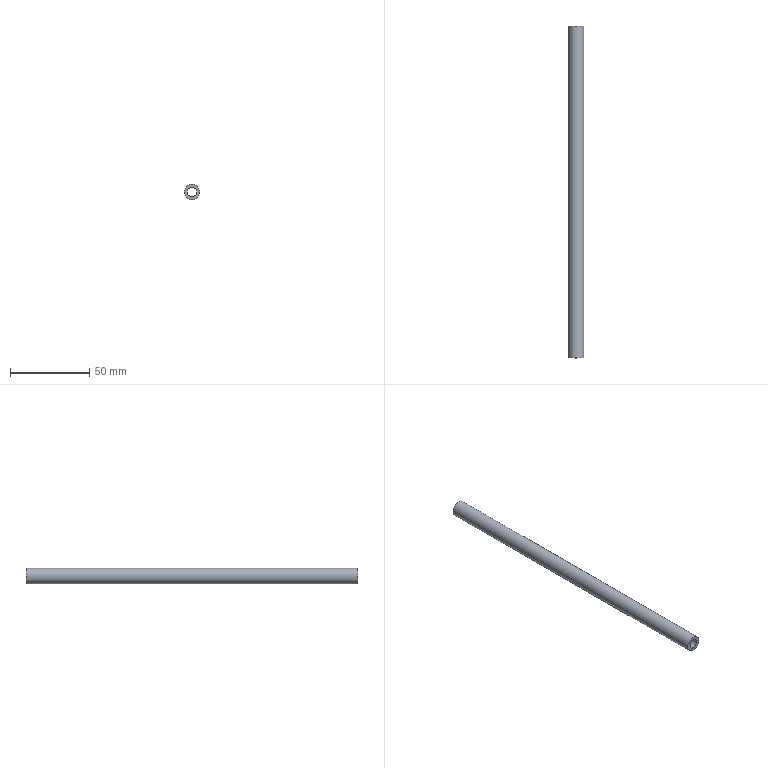Component | NX | CH3404_4-2 | 1 solid | 4 faces | box 10 x 210 x 10 mm | volume 10556 mm3 | cylinder 2 | plane 2 | commonest cylinder face diameters 10 x1 6 x1
STEP:
#1=CARTESIAN_POINT('',(0.,0.,0.));
#2=DIRECTION('',(0.,0.,1.));
#3=DIRECTION('',(1.,0.,0.));
#4=AXIS2_PLACEMENT_3D('',#1,#2,#3);
#5=CARTESIAN_POINT('',(5.,-18.,0.));
#6=VERTEX_POINT('',#5);
#7=CARTESIAN_POINT('',(0.,-18.,0.));
#8=DIRECTION('',(0.,-1.,0.));
#9=DIRECTION('',(1.,0.,0.));
#10=AXIS2_PLACEMENT_3D('',#7,#8,#9);
#11=CIRCLE('',#10,5.);
#12=CARTESIAN_POINT('',(0.,-18.,0.));
#13=DIRECTION('',(0.,1.,0.));
#14=DIRECTION('',(-1.,0.,0.));
#15=AXIS2_PLACEMENT_3D('',#12,#13,#14);
#16=CYLINDRICAL_SURFACE('',#15,5.);
#17=CARTESIAN_POINT('',(9.425,0.));
#18=DIRECTION('',(-1.,0.));
#19=VECTOR('',#18,1.);
#20=LINE('',#17,#19);
#21=(GEOMETRIC_REPRESENTATION_CONTEXT(2)PARAMETRIC_REPRESENTATION_CONTEXT()REPRESENTATION_CONTEXT('',''));
#22=DEFINITIONAL_REPRESENTATION('',(#20),#21);
#23=PCURVE('',#16,#22);
#24=CARTESIAN_POINT('',(0.,-18.,0.));
#25=DIRECTION('',(0.,-1.,0.));
#26=DIRECTION('',(1.,0.,0.));
#27=AXIS2_PLACEMENT_3D('',#24,#25,#26);
#28=PLANE('',#27);
#29=CARTESIAN_POINT('',(0.,0.));
#30=DIRECTION('',(1.,0.));
#31=AXIS2_PLACEMENT_2D('',#29,#30);
#32=CIRCLE('',#31,5.);
#33=(GEOMETRIC_REPRESENTATION_CONTEXT(2)PARAMETRIC_REPRESENTATION_CONTEXT()REPRESENTATION_CONTEXT('',''));
#34=DEFINITIONAL_REPRESENTATION('',(#32),#33);
#35=PCURVE('',#28,#34);
#36=SURFACE_CURVE('',#11,(#23,#35),.PCURVE_S1.);
#37=EDGE_CURVE('',#6,#6,#36,.T.);
#38=ORIENTED_EDGE('',*,*,#37,.F.);
#39=CARTESIAN_POINT('',(5.,192.,0.));
#40=VERTEX_POINT('',#39);
#41=CARTESIAN_POINT('',(5.,-18.,0.));
#42=CARTESIAN_POINT('',(5.,192.,0.));
#43=B_SPLINE_CURVE_WITH_KNOTS('',1,(#41,#42),.UNSPECIFIED.,.F.,.F.,(2,2),(0.,210.),.PIECEWISE_BEZIER_KNOTS.);
#44=CARTESIAN_POINT('',(9.425,0.));
#45=DIRECTION('',(0.,1.));
#46=VECTOR('',#45,1.);
#47=LINE('',#44,#46);
#48=(GEOMETRIC_REPRESENTATION_CONTEXT(2)PARAMETRIC_REPRESENTATION_CONTEXT()REPRESENTATION_CONTEXT('',''));
#49=DEFINITIONAL_REPRESENTATION('',(#47),#48);
#50=PCURVE('',#16,#49);
#51=CARTESIAN_POINT('',(3.142,0.));
#52=DIRECTION('',(0.,1.));
#53=VECTOR('',#52,1.);
#54=LINE('',#51,#53);
#55=(GEOMETRIC_REPRESENTATION_CONTEXT(2)PARAMETRIC_REPRESENTATION_CONTEXT()REPRESENTATION_CONTEXT('',''));
#56=DEFINITIONAL_REPRESENTATION('',(#54),#55);
#57=PCURVE('',#16,#56);
#58=SEAM_CURVE('',#43,(#50,#57),.PCURVE_S1.);
#59=EDGE_CURVE('',#6,#40,#58,.T.);
#60=ORIENTED_EDGE('',*,*,#59,.T.);
#61=CARTESIAN_POINT('',(0.,192.,0.));
#62=DIRECTION('',(0.,-1.,0.));
#63=DIRECTION('',(1.,0.,0.));
#64=AXIS2_PLACEMENT_3D('',#61,#62,#63);
#65=CIRCLE('',#64,5.);
#66=CARTESIAN_POINT('',(9.425,210.));
#67=DIRECTION('',(-1.,0.));
#68=VECTOR('',#67,1.);
#69=LINE('',#66,#68);
#70=(GEOMETRIC_REPRESENTATION_CONTEXT(2)PARAMETRIC_REPRESENTATION_CONTEXT()REPRESENTATION_CONTEXT('',''));
#71=DEFINITIONAL_REPRESENTATION('',(#69),#70);
#72=PCURVE('',#16,#71);
#73=CARTESIAN_POINT('',(0.,192.,0.));
#74=DIRECTION('',(0.,-1.,0.));
#75=DIRECTION('',(1.,0.,0.));
#76=AXIS2_PLACEMENT_3D('',#73,#74,#75);
#77=PLANE('',#76);
#78=CARTESIAN_POINT('',(0.,0.));
#79=DIRECTION('',(1.,0.));
#80=AXIS2_PLACEMENT_2D('',#78,#79);
#81=CIRCLE('',#80,5.);
#82=(GEOMETRIC_REPRESENTATION_CONTEXT(2)PARAMETRIC_REPRESENTATION_CONTEXT()REPRESENTATION_CONTEXT('',''));
#83=DEFINITIONAL_REPRESENTATION('',(#81),#82);
#84=PCURVE('',#77,#83);
#85=SURFACE_CURVE('',#65,(#72,#84),.PCURVE_S1.);
#86=EDGE_CURVE('',#40,#40,#85,.T.);
#87=ORIENTED_EDGE('',*,*,#86,.T.);
#88=ORIENTED_EDGE('',*,*,#59,.F.);
#89=EDGE_LOOP('',(#38,#60,#87,#88));
#90=FACE_BOUND('',#89,.T.);
#91=ADVANCED_FACE('',(#90),#16,.T.);
#92=CARTESIAN_POINT('',(3.,-18.,0.));
#93=VERTEX_POINT('',#92);
#94=CARTESIAN_POINT('',(0.,-18.,0.));
#95=DIRECTION('',(0.,-1.,0.));
#96=DIRECTION('',(1.,0.,0.));
#97=AXIS2_PLACEMENT_3D('',#94,#95,#96);
#98=CIRCLE('',#97,3.);
#99=CARTESIAN_POINT('',(0.,-18.,0.));
#100=DIRECTION('',(0.,1.,0.));
#101=DIRECTION('',(-1.,0.,0.));
#102=AXIS2_PLACEMENT_3D('',#99,#100,#101);
#103=CYLINDRICAL_SURFACE('',#102,3.);
#104=CARTESIAN_POINT('',(9.425,0.));
#105=DIRECTION('',(-1.,0.));
#106=VECTOR('',#105,1.);
#107=LINE('',#104,#106);
#108=(GEOMETRIC_REPRESENTATION_CONTEXT(2)PARAMETRIC_REPRESENTATION_CONTEXT()REPRESENTATION_CONTEXT('',''));
#109=DEFINITIONAL_REPRESENTATION('',(#107),#108);
#110=PCURVE('',#103,#109);
#111=CARTESIAN_POINT('',(0.,0.));
#112=DIRECTION('',(1.,0.));
#113=AXIS2_PLACEMENT_2D('',#111,#112);
#114=CIRCLE('',#113,3.);
#115=(GEOMETRIC_REPRESENTATION_CONTEXT(2)PARAMETRIC_REPRESENTATION_CONTEXT()REPRESENTATION_CONTEXT('',''));
#116=DEFINITIONAL_REPRESENTATION('',(#114),#115);
#117=PCURVE('',#28,#116);
#118=SURFACE_CURVE('',#98,(#110,#117),.PCURVE_S1.);
#119=EDGE_CURVE('',#93,#93,#118,.T.);
#120=ORIENTED_EDGE('',*,*,#119,.F.);
#121=CARTESIAN_POINT('',(3.,192.,0.));
#122=VERTEX_POINT('',#121);
#123=CARTESIAN_POINT('',(3.,-18.,0.));
#124=CARTESIAN_POINT('',(3.,192.,0.));
#125=B_SPLINE_CURVE_WITH_KNOTS('',1,(#123,#124),.UNSPECIFIED.,.F.,.F.,(2,2),(0.,210.),.PIECEWISE_BEZIER_KNOTS.);
#126=CARTESIAN_POINT('',(9.425,0.));
#127=DIRECTION('',(0.,1.));
#128=VECTOR('',#127,1.);
#129=LINE('',#126,#128);
#130=(GEOMETRIC_REPRESENTATION_CONTEXT(2)PARAMETRIC_REPRESENTATION_CONTEXT()REPRESENTATION_CONTEXT('',''));
#131=DEFINITIONAL_REPRESENTATION('',(#129),#130);
#132=PCURVE('',#103,#131);
#133=CARTESIAN_POINT('',(3.142,0.));
#134=DIRECTION('',(0.,1.));
#135=VECTOR('',#134,1.);
#136=LINE('',#133,#135);
#137=(GEOMETRIC_REPRESENTATION_CONTEXT(2)PARAMETRIC_REPRESENTATION_CONTEXT()REPRESENTATION_CONTEXT('',''));
#138=DEFINITIONAL_REPRESENTATION('',(#136),#137);
#139=PCURVE('',#103,#138);
#140=SEAM_CURVE('',#125,(#132,#139),.PCURVE_S1.);
#141=EDGE_CURVE('',#93,#122,#140,.T.);
#142=ORIENTED_EDGE('',*,*,#141,.T.);
#143=CARTESIAN_POINT('',(0.,192.,0.));
#144=DIRECTION('',(0.,-1.,0.));
#145=DIRECTION('',(1.,0.,0.));
#146=AXIS2_PLACEMENT_3D('',#143,#144,#145);
#147=CIRCLE('',#146,3.);
#148=CARTESIAN_POINT('',(9.425,210.));
#149=DIRECTION('',(-1.,0.));
#150=VECTOR('',#149,1.);
#151=LINE('',#148,#150);
#152=(GEOMETRIC_REPRESENTATION_CONTEXT(2)PARAMETRIC_REPRESENTATION_CONTEXT()REPRESENTATION_CONTEXT('',''));
#153=DEFINITIONAL_REPRESENTATION('',(#151),#152);
#154=PCURVE('',#103,#153);
#155=CARTESIAN_POINT('',(0.,0.));
#156=DIRECTION('',(1.,0.));
#157=AXIS2_PLACEMENT_2D('',#155,#156);
#158=CIRCLE('',#157,3.);
#159=(GEOMETRIC_REPRESENTATION_CONTEXT(2)PARAMETRIC_REPRESENTATION_CONTEXT()REPRESENTATION_CONTEXT('',''));
#160=DEFINITIONAL_REPRESENTATION('',(#158),#159);
#161=PCURVE('',#77,#160);
#162=SURFACE_CURVE('',#147,(#154,#161),.PCURVE_S1.);
#163=EDGE_CURVE('',#122,#122,#162,.T.);
#164=ORIENTED_EDGE('',*,*,#163,.T.);
#165=ORIENTED_EDGE('',*,*,#141,.F.);
#166=EDGE_LOOP('',(#120,#142,#164,#165));
#167=FACE_BOUND('',#166,.F.);
#168=ADVANCED_FACE('',(#167),#103,.F.);
#169=ORIENTED_EDGE('',*,*,#37,.T.);
#170=EDGE_LOOP('',(#169));
#171=FACE_BOUND('',#170,.T.);
#172=ORIENTED_EDGE('',*,*,#119,.F.);
#173=EDGE_LOOP('',(#172));
#174=FACE_BOUND('',#173,.T.);
#175=ADVANCED_FACE('',(#171,#174),#28,.T.);
#176=ORIENTED_EDGE('',*,*,#86,.F.);
#177=EDGE_LOOP('',(#176));
#178=FACE_BOUND('',#177,.T.);
#179=ORIENTED_EDGE('',*,*,#163,.T.);
#180=EDGE_LOOP('',(#179));
#181=FACE_BOUND('',#180,.T.);
#182=ADVANCED_FACE('',(#178,#181),#77,.F.);
#183=CLOSED_SHELL('',(#91,#168,#175,#182));
#184=MANIFOLD_SOLID_BREP('',#183);
#185=(LENGTH_UNIT()NAMED_UNIT(*)SI_UNIT(.MILLI.,.METRE.));
#186=UNCERTAINTY_MEASURE_WITH_UNIT(LENGTH_MEASURE(0.00001),#185,'','');
#187=(NAMED_UNIT(*)PLANE_ANGLE_UNIT()SI_UNIT($,.RADIAN.));
#188=(NAMED_UNIT(*)SI_UNIT($,.STERADIAN.)SOLID_ANGLE_UNIT());
#189=(GEOMETRIC_REPRESENTATION_CONTEXT(3)GLOBAL_UNCERTAINTY_ASSIGNED_CONTEXT((#186))GLOBAL_UNIT_ASSIGNED_CONTEXT((#185,#187,#188))REPRESENTATION_CONTEXT('',''));
#190=ADVANCED_BREP_SHAPE_REPRESENTATION('',(#4,#184),#189);